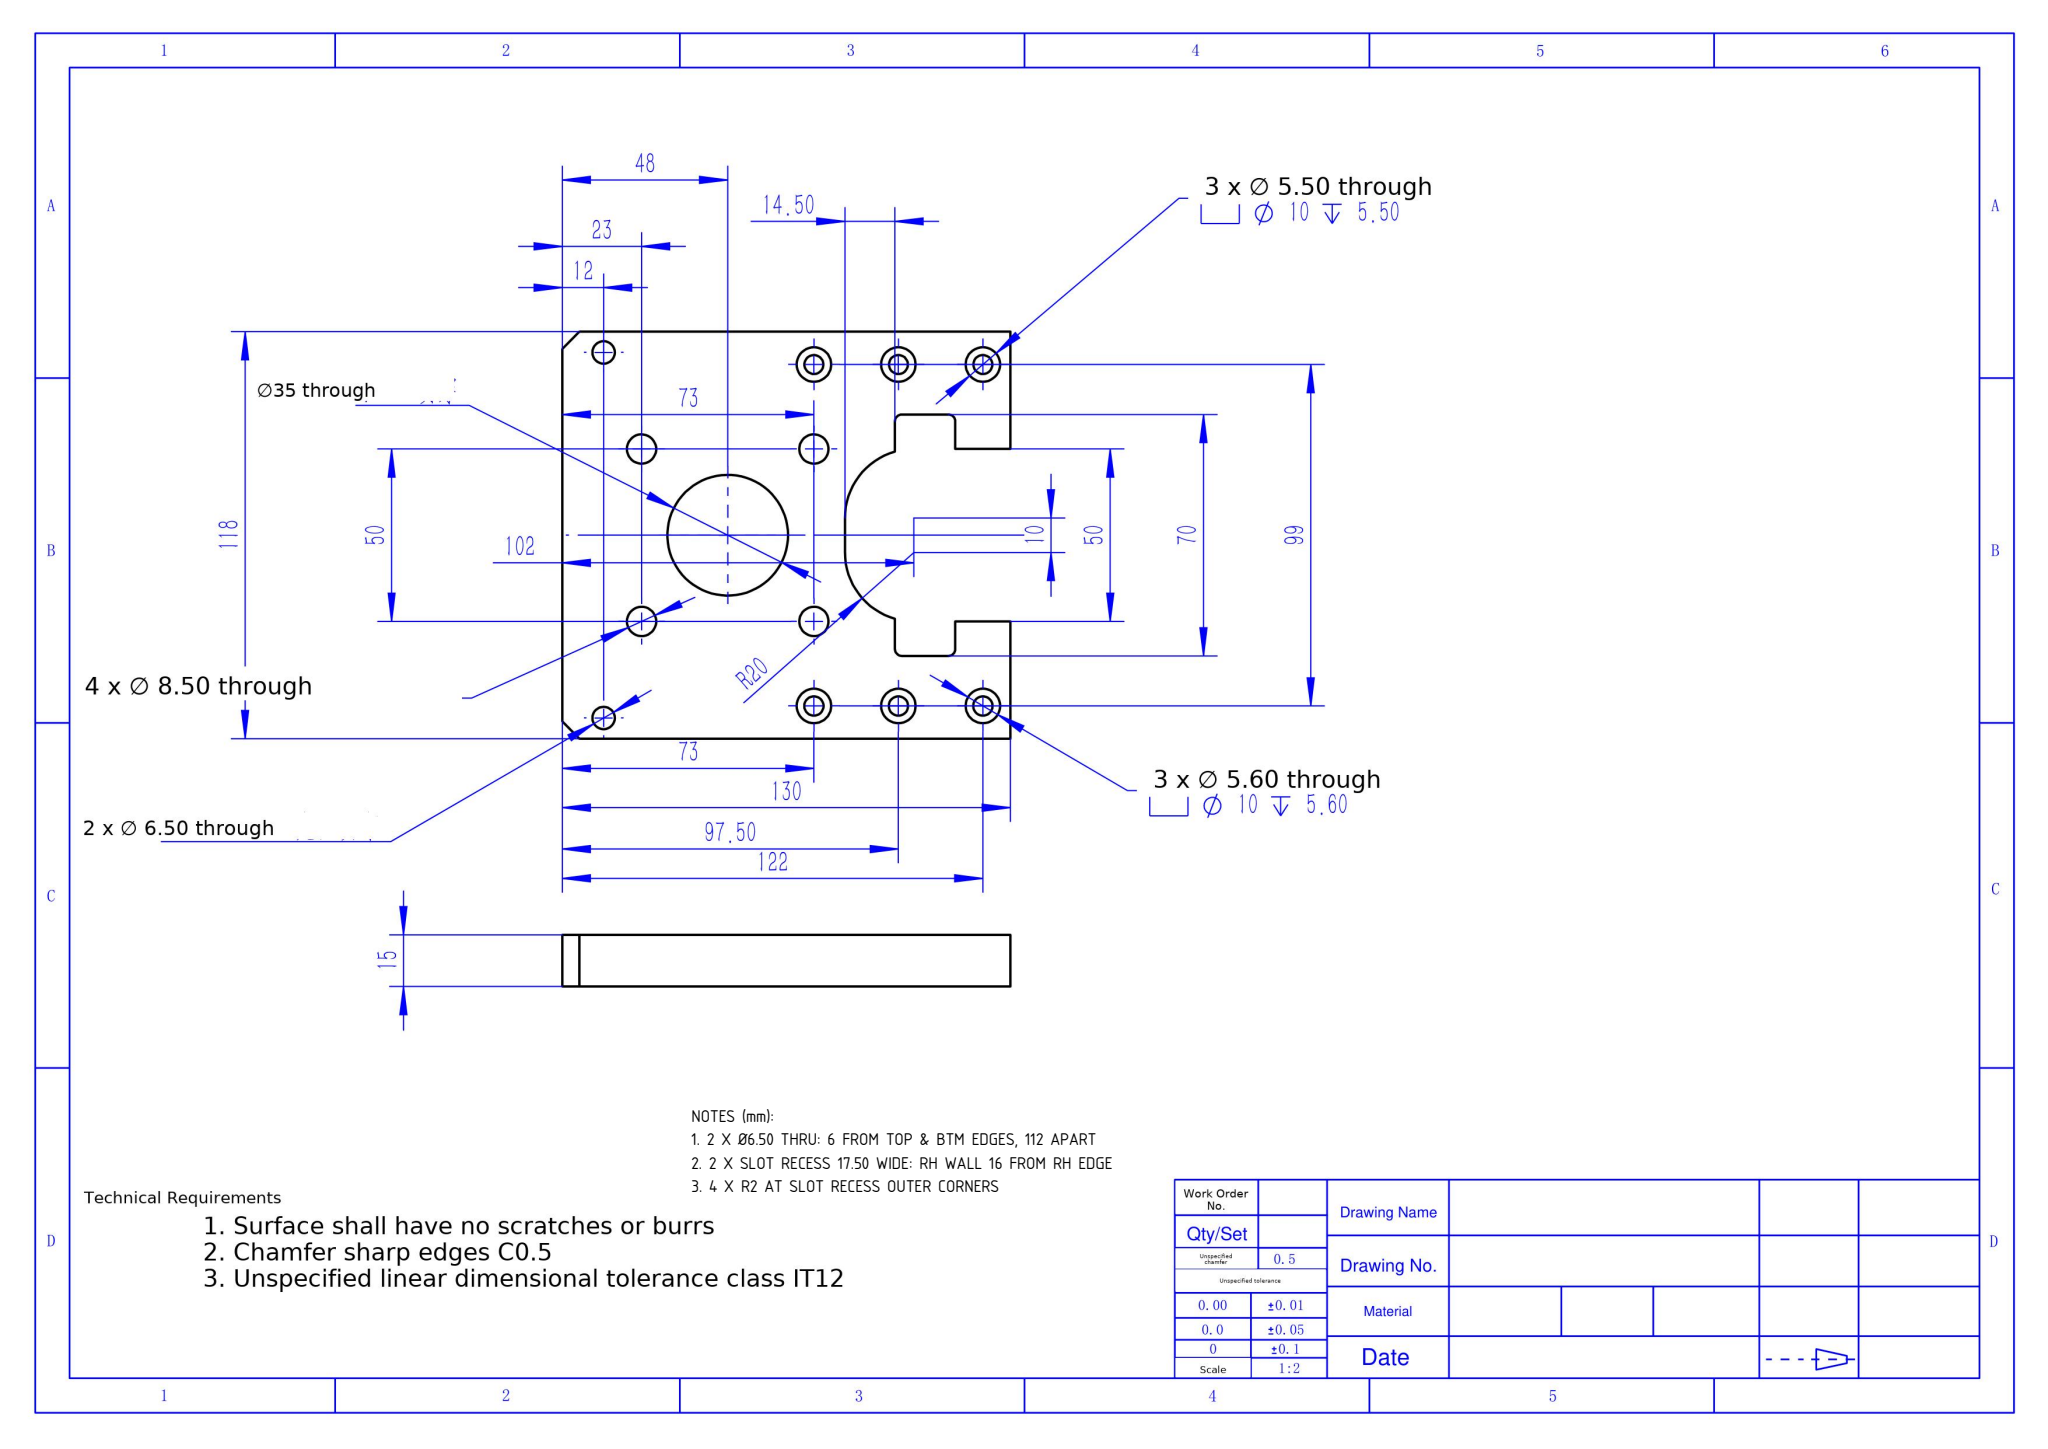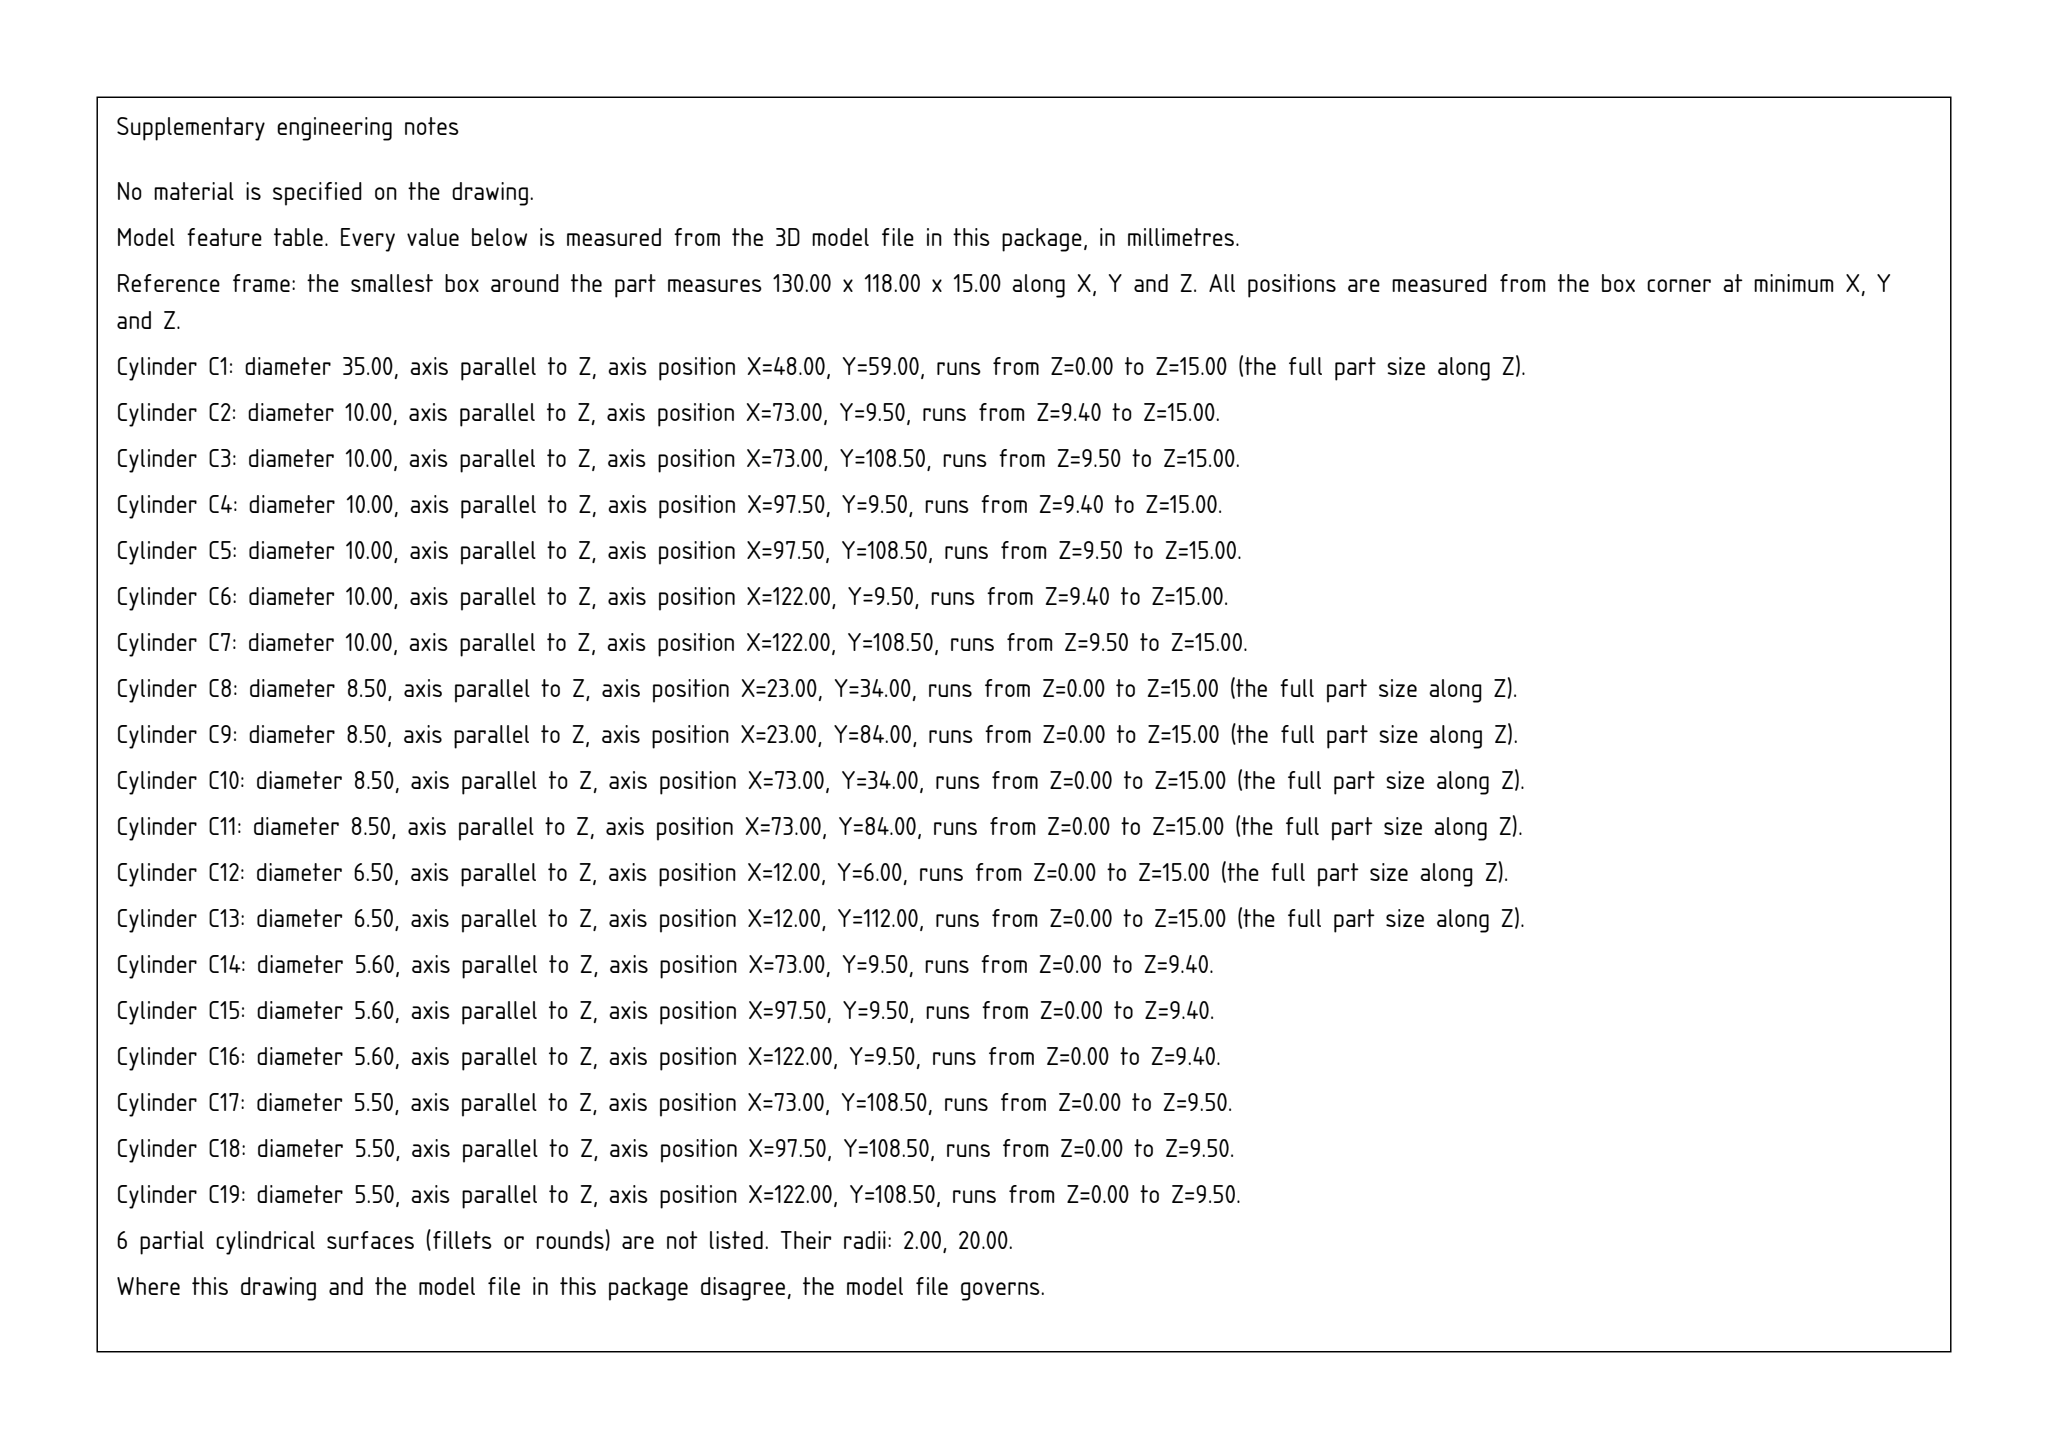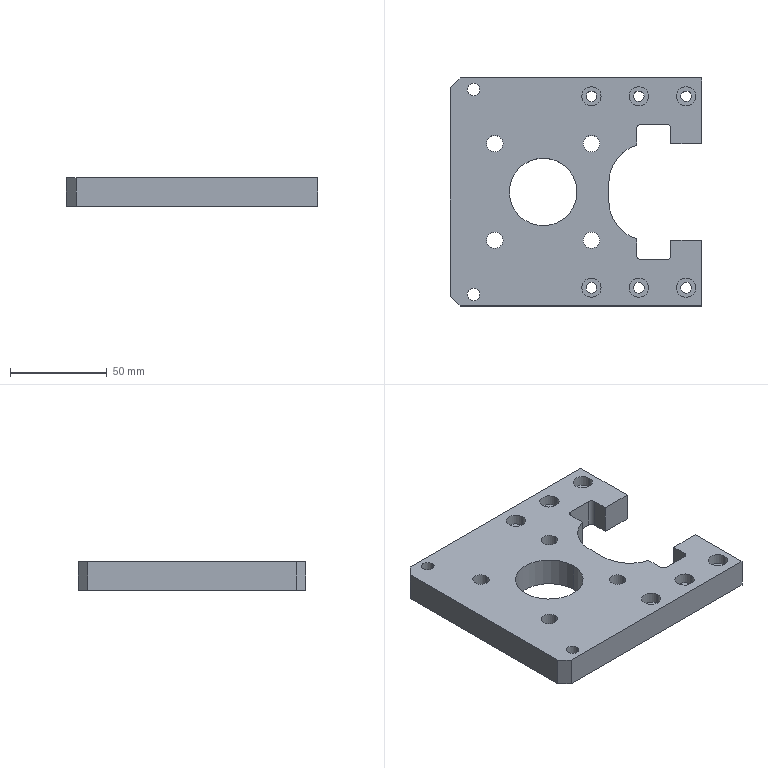Part | SolidWorks | mm | 1 solid | 68 faces | box 130 x 118 x 15 mm | volume 168241 mm3 | cylinder 44 | plane 24 | commonest cylinder face diameters 10 x12 8.5 x8 5.6 x6 5.5 x6 6.5 x4 4 x4 35 x2 40 x2
Drawing notes:
2 X Ø6.50 THRU: 6 FROM TOP & BTM EDGES, 112 APART | from the solid: Ø6.5 z-cyls at (12,6) and (12,112); bbox Y=118 -> 6 from each edge
2 X SLOT RECESS 17.50 WIDE: RH WALL 16 FROM RH EDGE | from the solid: x-planes at 96.5 and 114; 114-96.5=17.5; bbox X=130 -> 130-114=16
4 X R2 AT SLOT RECESS OUTER CORNERS | from the solid: Ø4 z-cyls at (98.5,26),(112,26),(98.5,92),(112,92) tangent to x=96.5/114, y=24/94
build123d program:
from build123d import *

# Parameters (mm, degrees)
SKETCH1_W                                            = 130
SKETCH1_H                                            = 118
BOSS_EXTRUDE1_DEPTH                                  = 15
SKETCH2_W                                            = 96
SKETCH2_H                                            = 50
CUT_EXTRUDE1_DEPTH                                   = 177.207
FILLET1_R                                            = 20
SKETCH3_R                                            = 17.5
CUT_EXTRUDE2_DEPTH                                   = 177.207
F_8_5_8_5_DIAMETER_HOLE1_D                           = 8.5
M5_HEX_HEAD_BOLT_CYLINDRICAL_COUNTERSUNK_D           = 5.5
M5_HEX_HEAD_BOLT_CYLINDRICAL_COUNTERSUNK_CBORE_D     = 10
M5_HEX_HEAD_BOLT_CYLINDRICAL_COUNTERSUNK_CBORE_DEPTH = 5.5
SKETCH8_W                                            = 17.5
SKETCH8_H                                            = 20
CUT_EXTRUDE3_DEPTH                                   = 177.207
FILLET2_R                                            = 2
CHAMFER1_SIZE                                        = 5
M5_HEX_HEAD_BOLT_CYLINDRICAL_COUNTER_2_D             = 5.6
M5_HEX_HEAD_BOLT_CYLINDRICAL_COUNTER_2_CBORE_D       = 10
M5_HEX_HEAD_BOLT_CYLINDRICAL_COUNTER_2_CBORE_DEPTH   = 5.6
F_6_5_6_5_DIAMETER_HOLE1_D                           = 6.5


with BuildPart() as part:
    # Sketch1 → Boss-Extrude1 (new body)
    with BuildSketch(Plane.XY):
        with Locations((65, 59)):
            Rectangle(SKETCH1_W, SKETCH1_H)
    extrude(amount=BOSS_EXTRUDE1_DEPTH)

    # Sketch2 → Cut-Extrude1 (cut, through all)
    with BuildSketch(Plane.XY.offset(15)):
        with Locations((130, 59)):
            Rectangle(SKETCH2_W, SKETCH2_H)
    extrude(amount=-CUT_EXTRUDE1_DEPTH, mode=Mode.SUBTRACT)

    # Fillet1
    fillet1_edges = [part.edges().sort_by_distance(p)[0] for p in [
        (82, 84, 7.5),
        (82, 34, 7.5),
    ]]
    fillet(fillet1_edges, radius=FILLET1_R)

    # Sketch3 → Cut-Extrude2 (cut, through all)
    with BuildSketch(Plane.XY.offset(15)):
        with Locations((48, 59)):
            Circle(SKETCH3_R)
    extrude(amount=-CUT_EXTRUDE2_DEPTH, mode=Mode.SUBTRACT)

    # 8.5 _8.5_ Diameter Hole1 (through all)
    with Locations(Plane(origin=(73, 84, 0), x_dir=(-1, 0, 0), z_dir=(0, 0, -1))):
        with Locations((0, 0), (50, 0), (0, -50), (50, -50)):
            Hole(F_8_5_8_5_DIAMETER_HOLE1_D / 2)

    # M5 Hex Head Bolt Cylindrical Countersunk (through all)
    with Locations(Plane(origin=(122, 108.5, 15), x_dir=(1, 0, 0), z_dir=(0, 0, 1))):
        with Locations((0, 0), (-24.5, 0), (-49, 0)):
            CounterBoreHole(M5_HEX_HEAD_BOLT_CYLINDRICAL_COUNTERSUNK_D / 2, M5_HEX_HEAD_BOLT_CYLINDRICAL_COUNTERSUNK_CBORE_D / 2, M5_HEX_HEAD_BOLT_CYLINDRICAL_COUNTERSUNK_CBORE_DEPTH)

    # Sketch8 → Cut-Extrude3 (cut, through all)
    with BuildSketch(Plane.XY.offset(15)):
        with Locations((105.25, 34)):
            Rectangle(SKETCH8_W, SKETCH8_H)
        with Locations((105.25, 84)):
            Rectangle(SKETCH8_W, SKETCH8_H)
    extrude(amount=-CUT_EXTRUDE3_DEPTH, mode=Mode.SUBTRACT)

    # Fillet2
    fillet2_edges = [part.edges().sort_by_distance(p)[0] for p in [
        (96.5, 24, 7.5),
        (114, 24, 7.5),
        (114, 94, 7.5),
        (96.5, 94, 7.5),
    ]]
    fillet(fillet2_edges, radius=FILLET2_R)

    # Chamfer1
    chamfer1_edges = [part.edges().sort_by_distance(p)[0] for p in [
        (0, 118, 7.5),
        (0, 0, 7.5),
    ]]
    chamfer(chamfer1_edges, length=CHAMFER1_SIZE)

    # M5 Hex Head Bolt Cylindrical Counter 2 (through all)
    with Locations(Plane(origin=(122, 9.5, 15), x_dir=(1, 0, 0), z_dir=(0, 0, 1))):
        with Locations((0, 0), (-24.5, 0), (-49, 0)):
            CounterBoreHole(M5_HEX_HEAD_BOLT_CYLINDRICAL_COUNTER_2_D / 2, M5_HEX_HEAD_BOLT_CYLINDRICAL_COUNTER_2_CBORE_D / 2, M5_HEX_HEAD_BOLT_CYLINDRICAL_COUNTER_2_CBORE_DEPTH)

    # 6.5 _6.5_ Diameter Hole1 (through all)
    with Locations(Plane(origin=(12, 112, 15), x_dir=(1, 0, 0), z_dir=(0, 0, 1))):
        with Locations((0, 0), (0, -106)):
            Hole(F_6_5_6_5_DIAMETER_HOLE1_D / 2)


solid = part.part